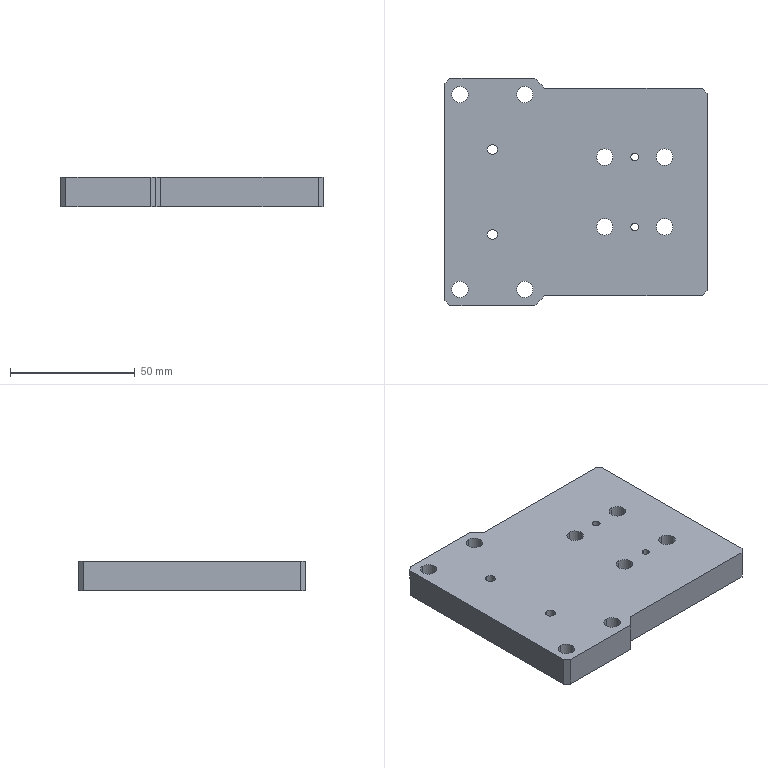Component | SolidWorks | AX.B92.SA.7371.18-2 | 1 solid | 64 faces | volume 101068 mm3 | cylinder 40 | plane 24 | commonest cylinder face diameters 11 x16 6.6 x16 3 x4 4 x4 | material 6061